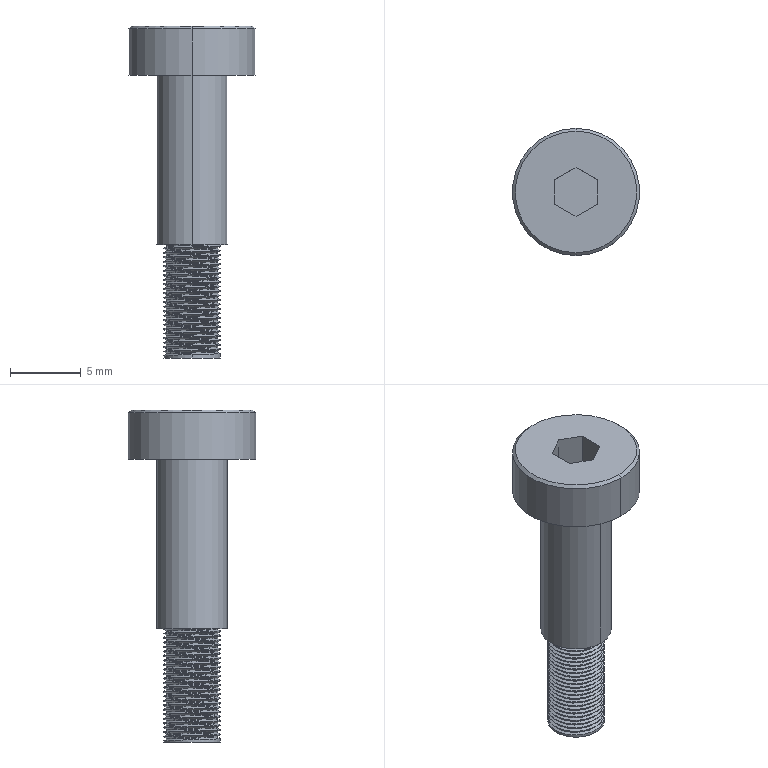Component | SolidWorks | SetScrewM4-D5-12-1 | 1 solid | 75 faces | volume 530 mm3 | cylinder 56 | plane 13 | spline 4 | cone 2 | commonest cylinder face diameters 4 x52 9 x2 5 x2